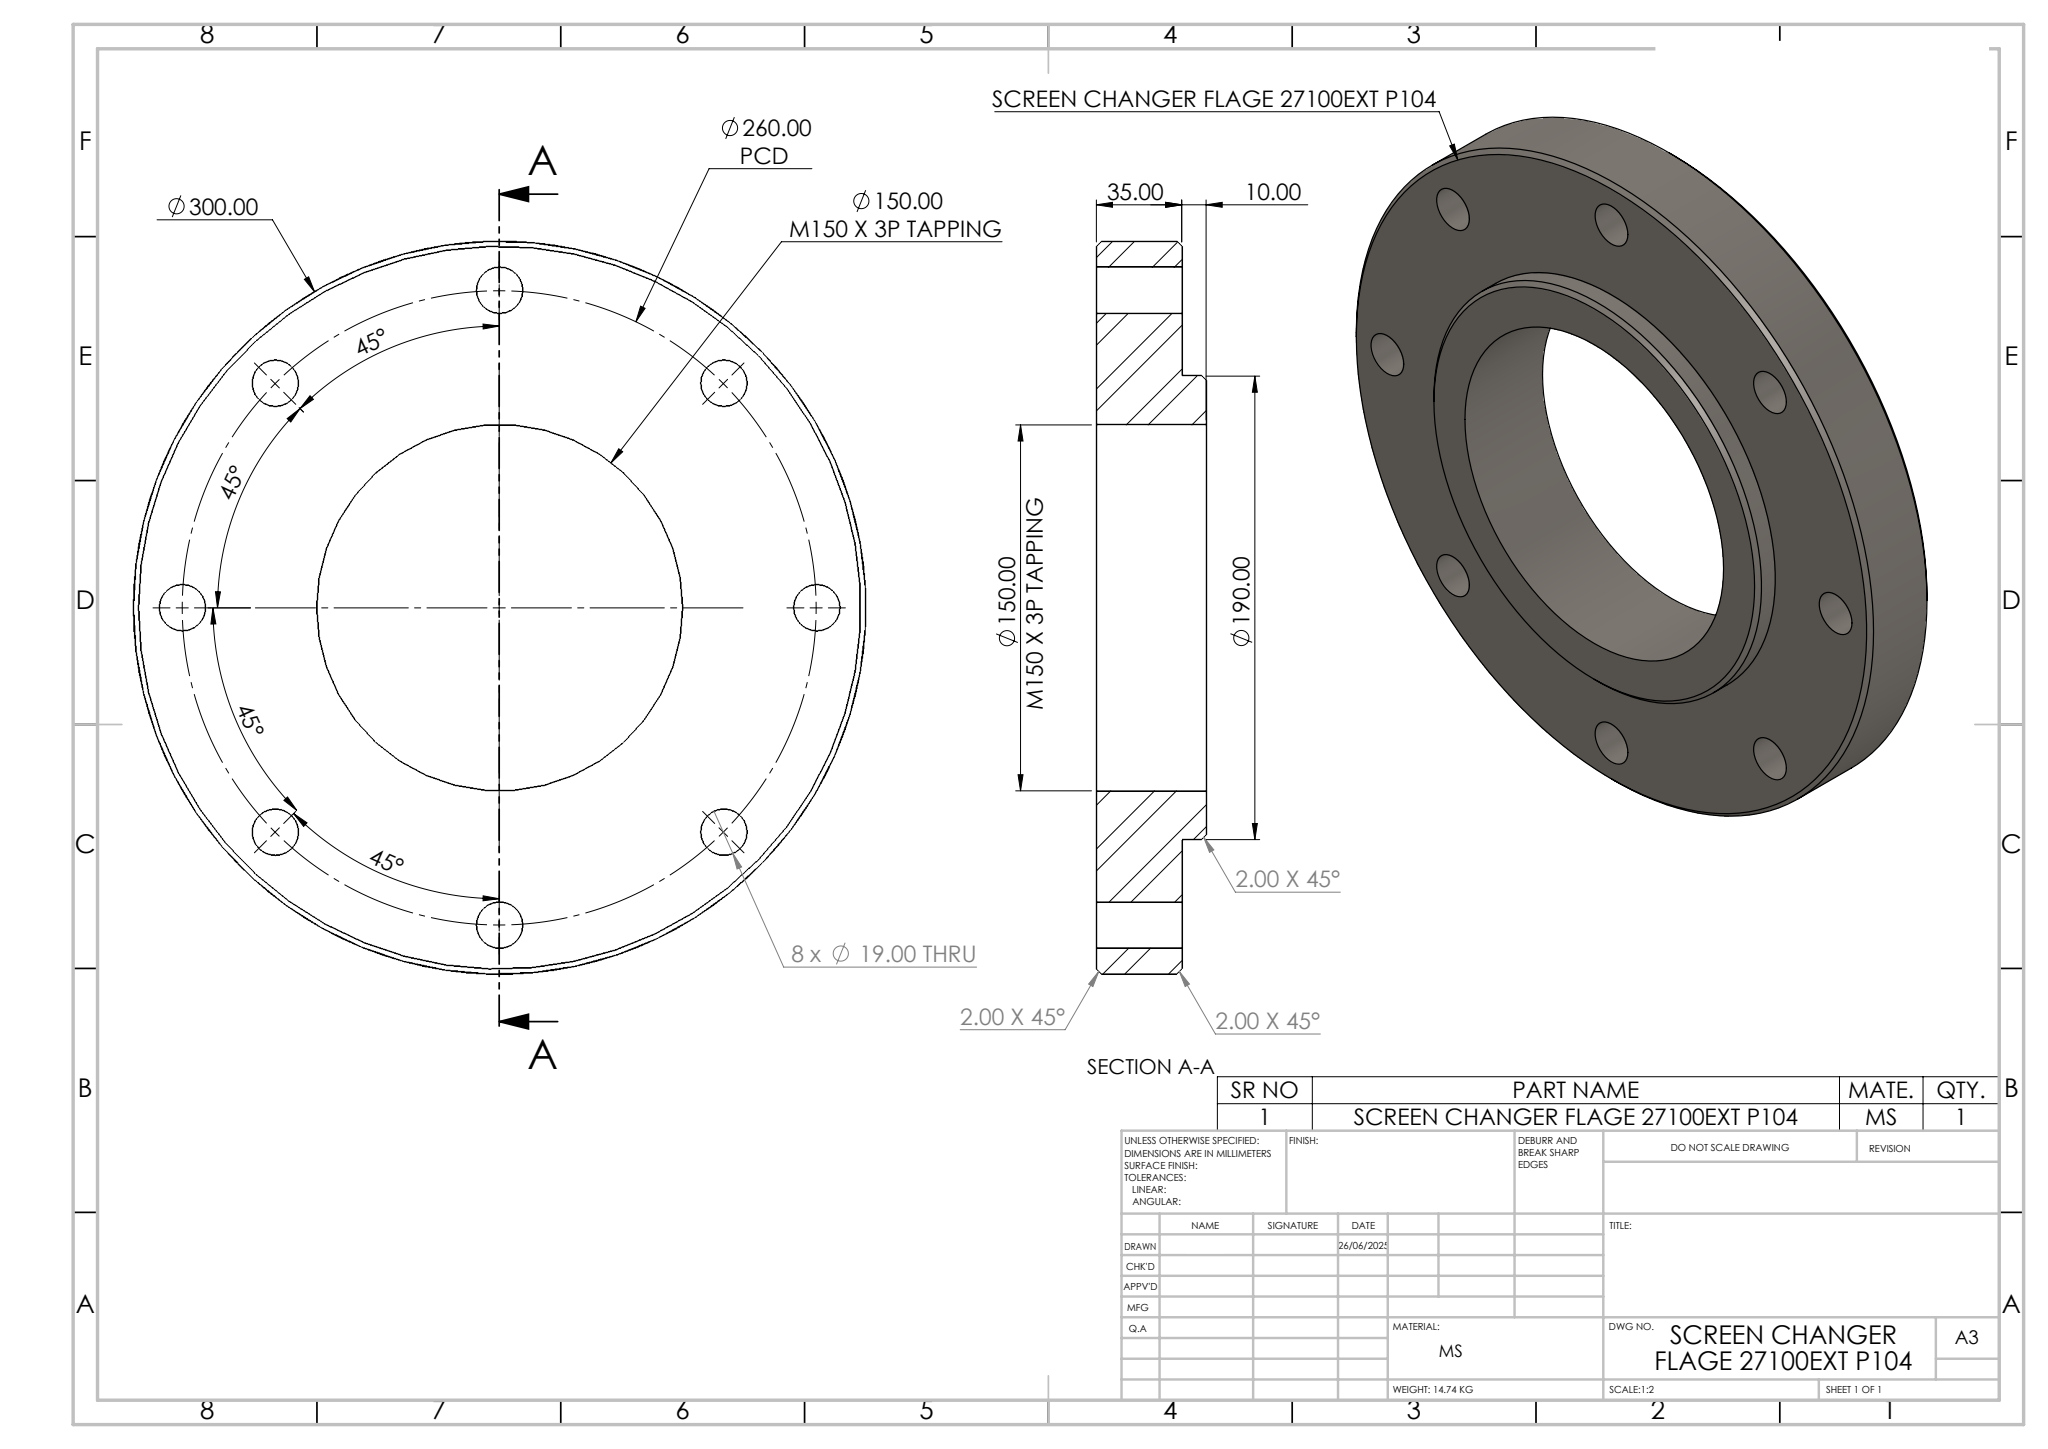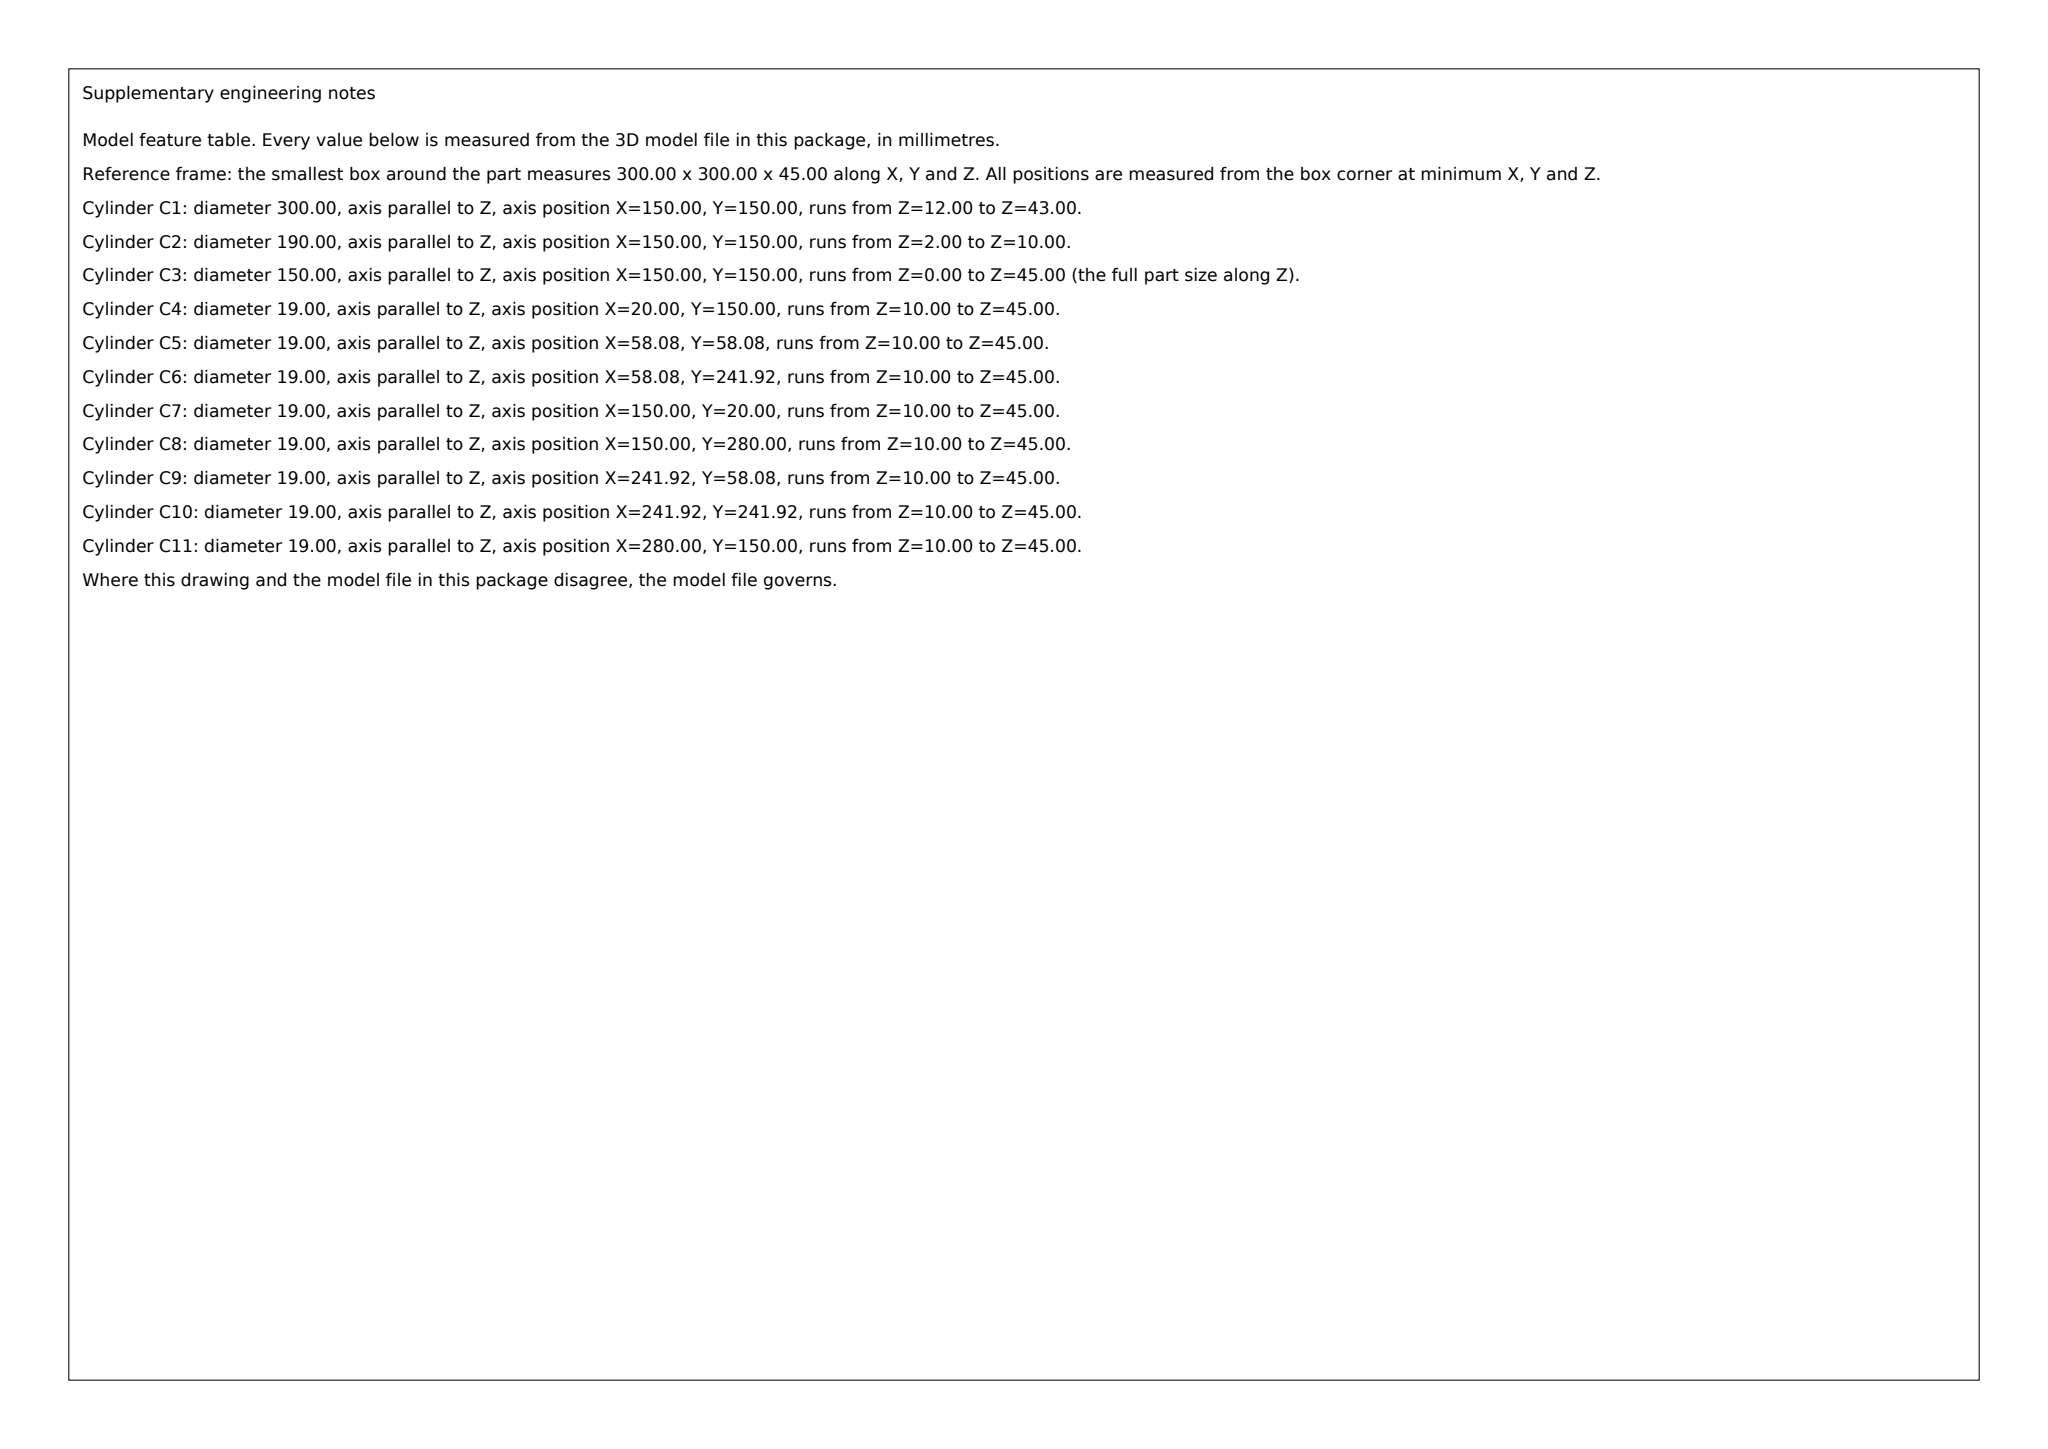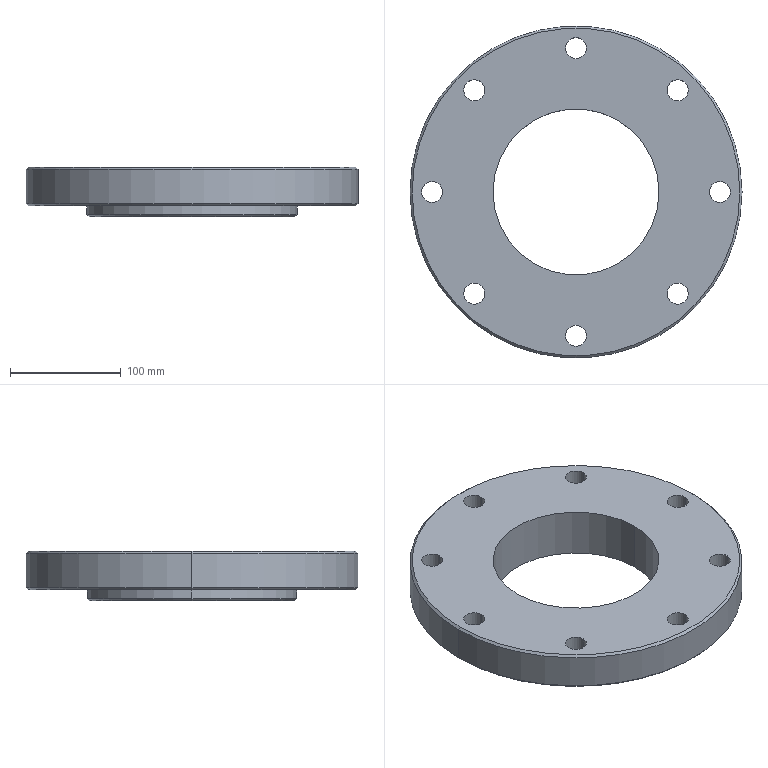Part | SolidWorks | mm | 1 solid | 31 faces | box 300 x 300 x 45 mm | volume 1877991 mm3 | cylinder 22 | cone 6 | plane 3 | commonest cylinder face diameters 19 x16 150 x2 300 x2 190 x2
build123d program:
from build123d import *

# Parameters (mm, degrees)
M16_CLEARANCE_HOLE1_D      = 19
CIRPATTERN1_COUNT          = 8
CHAMFER1_SIZE              = 2
F_1_0_150_DIAMETER_HOLE1_D = 150


with BuildPart() as part:
    # Sketch1 → Revolve1 (revolve)
    with BuildSketch(Plane(origin=(0, 0, 0), x_dir=(0, 0, -1), z_dir=(1, 0, 0)), mode=Mode.PRIVATE) as revolve1_sk:
        Polygon((0, 0), (0, 95), (-10, 95), (-10, 150), (-45, 150), (-45, 0), align=None)
    revolve(revolve1_sk.sketch.rotate(Axis((0, 0, 0), (0, 0, -1)), 90), axis=Axis((0, 0, 0), (0, 0, -1)))

    # M16 Clearance Hole1 (through all)
    with Locations(Plane(origin=(0, 0, 10), x_dir=(-1, 0, 0), z_dir=(0, 0, -1))):
        with Locations((0, 130)):
            m16_clearance_hole1 = Hole(M16_CLEARANCE_HOLE1_D / 2)

    # CirPattern1: M16 Clearance Hole1 ×8 about axis
    cirpattern1_axis = Axis((0, 0, 0), (0, 0, 1))
    for i in range(1, CIRPATTERN1_COUNT):
        add(m16_clearance_hole1.rotate(cirpattern1_axis, i * 360 / CIRPATTERN1_COUNT), mode=Mode.SUBTRACT)

    # Chamfer1
    chamfer1_edges = [part.edges().sort_by_distance(p)[0] for p in [
        (-150, 0, 10),
        (-150, 0, 45),
        (-95, 0, 0),
    ]]
    chamfer(chamfer1_edges, length=CHAMFER1_SIZE)

    # 1.0 _150_ Diameter Hole1 (through all)
    with Locations(Plane.XY.offset(45)):
        with Locations((0, 0)):
            Hole(F_1_0_150_DIAMETER_HOLE1_D / 2)


solid = part.part